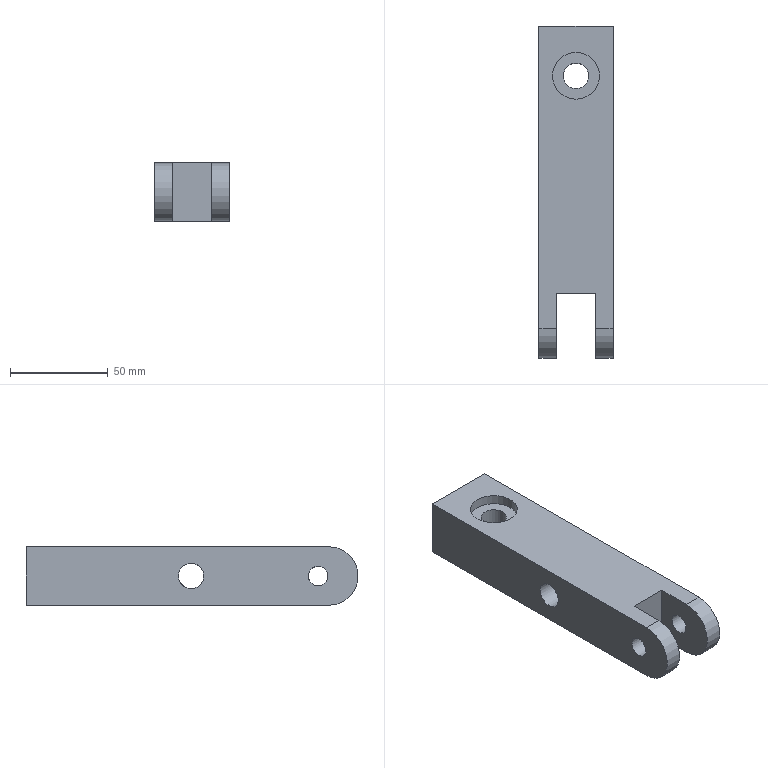Component | NX | CLAMP_PLATE | 1 solid | 22 faces | volume 131173 mm3 | plane 13 | cylinder 9 | commonest cylinder face diameters 13 x3 30 x2 10 x2 140 x1 24 x1